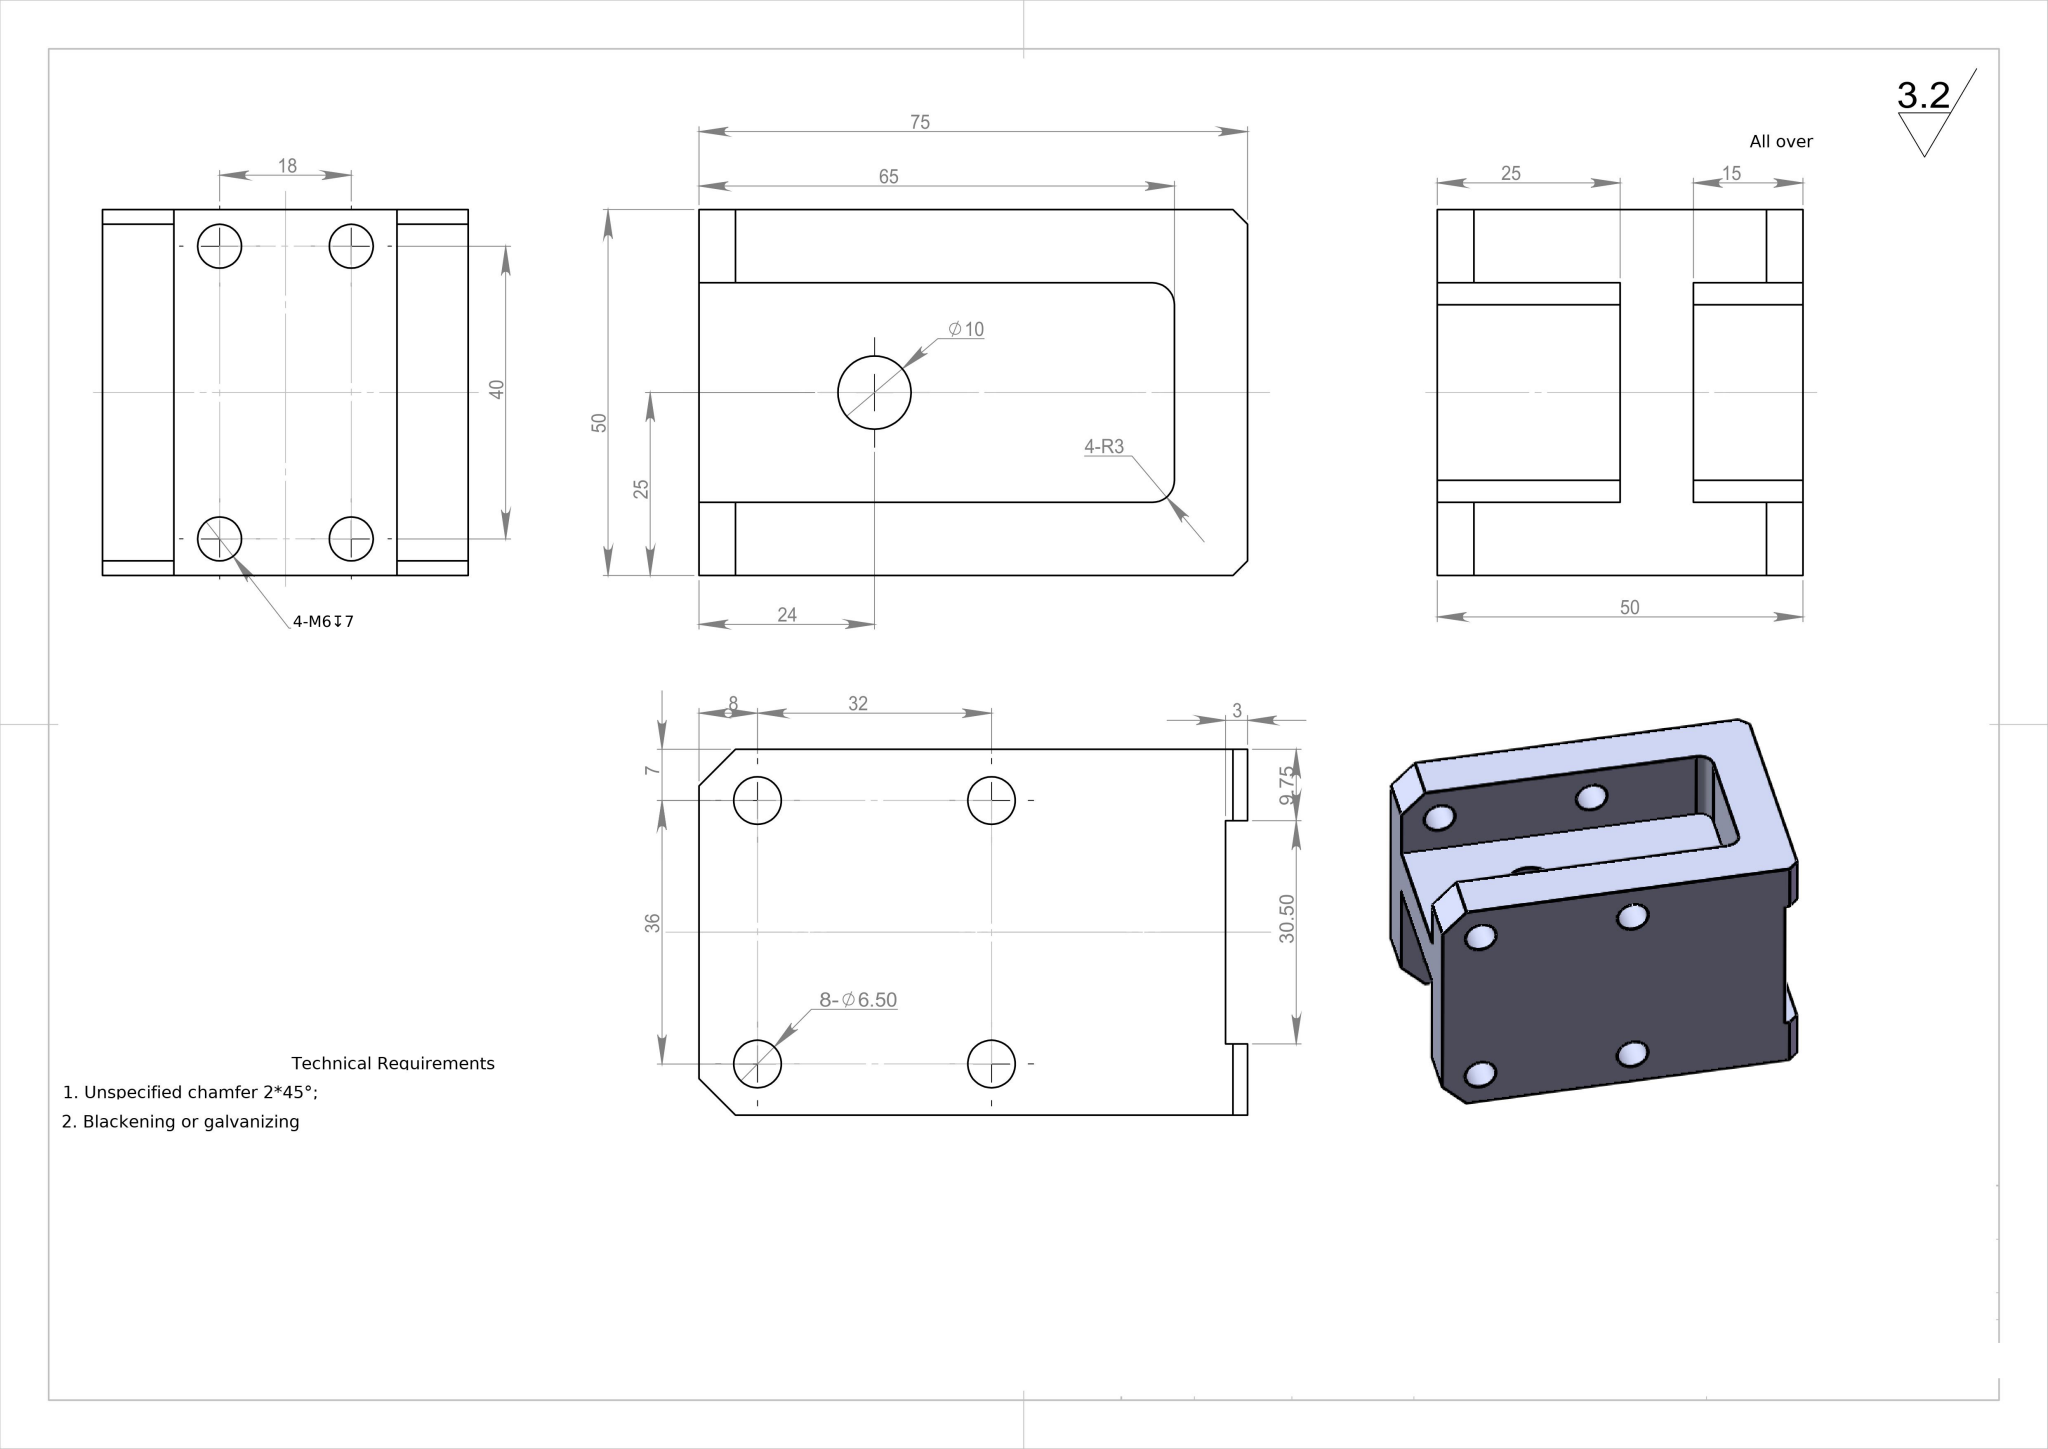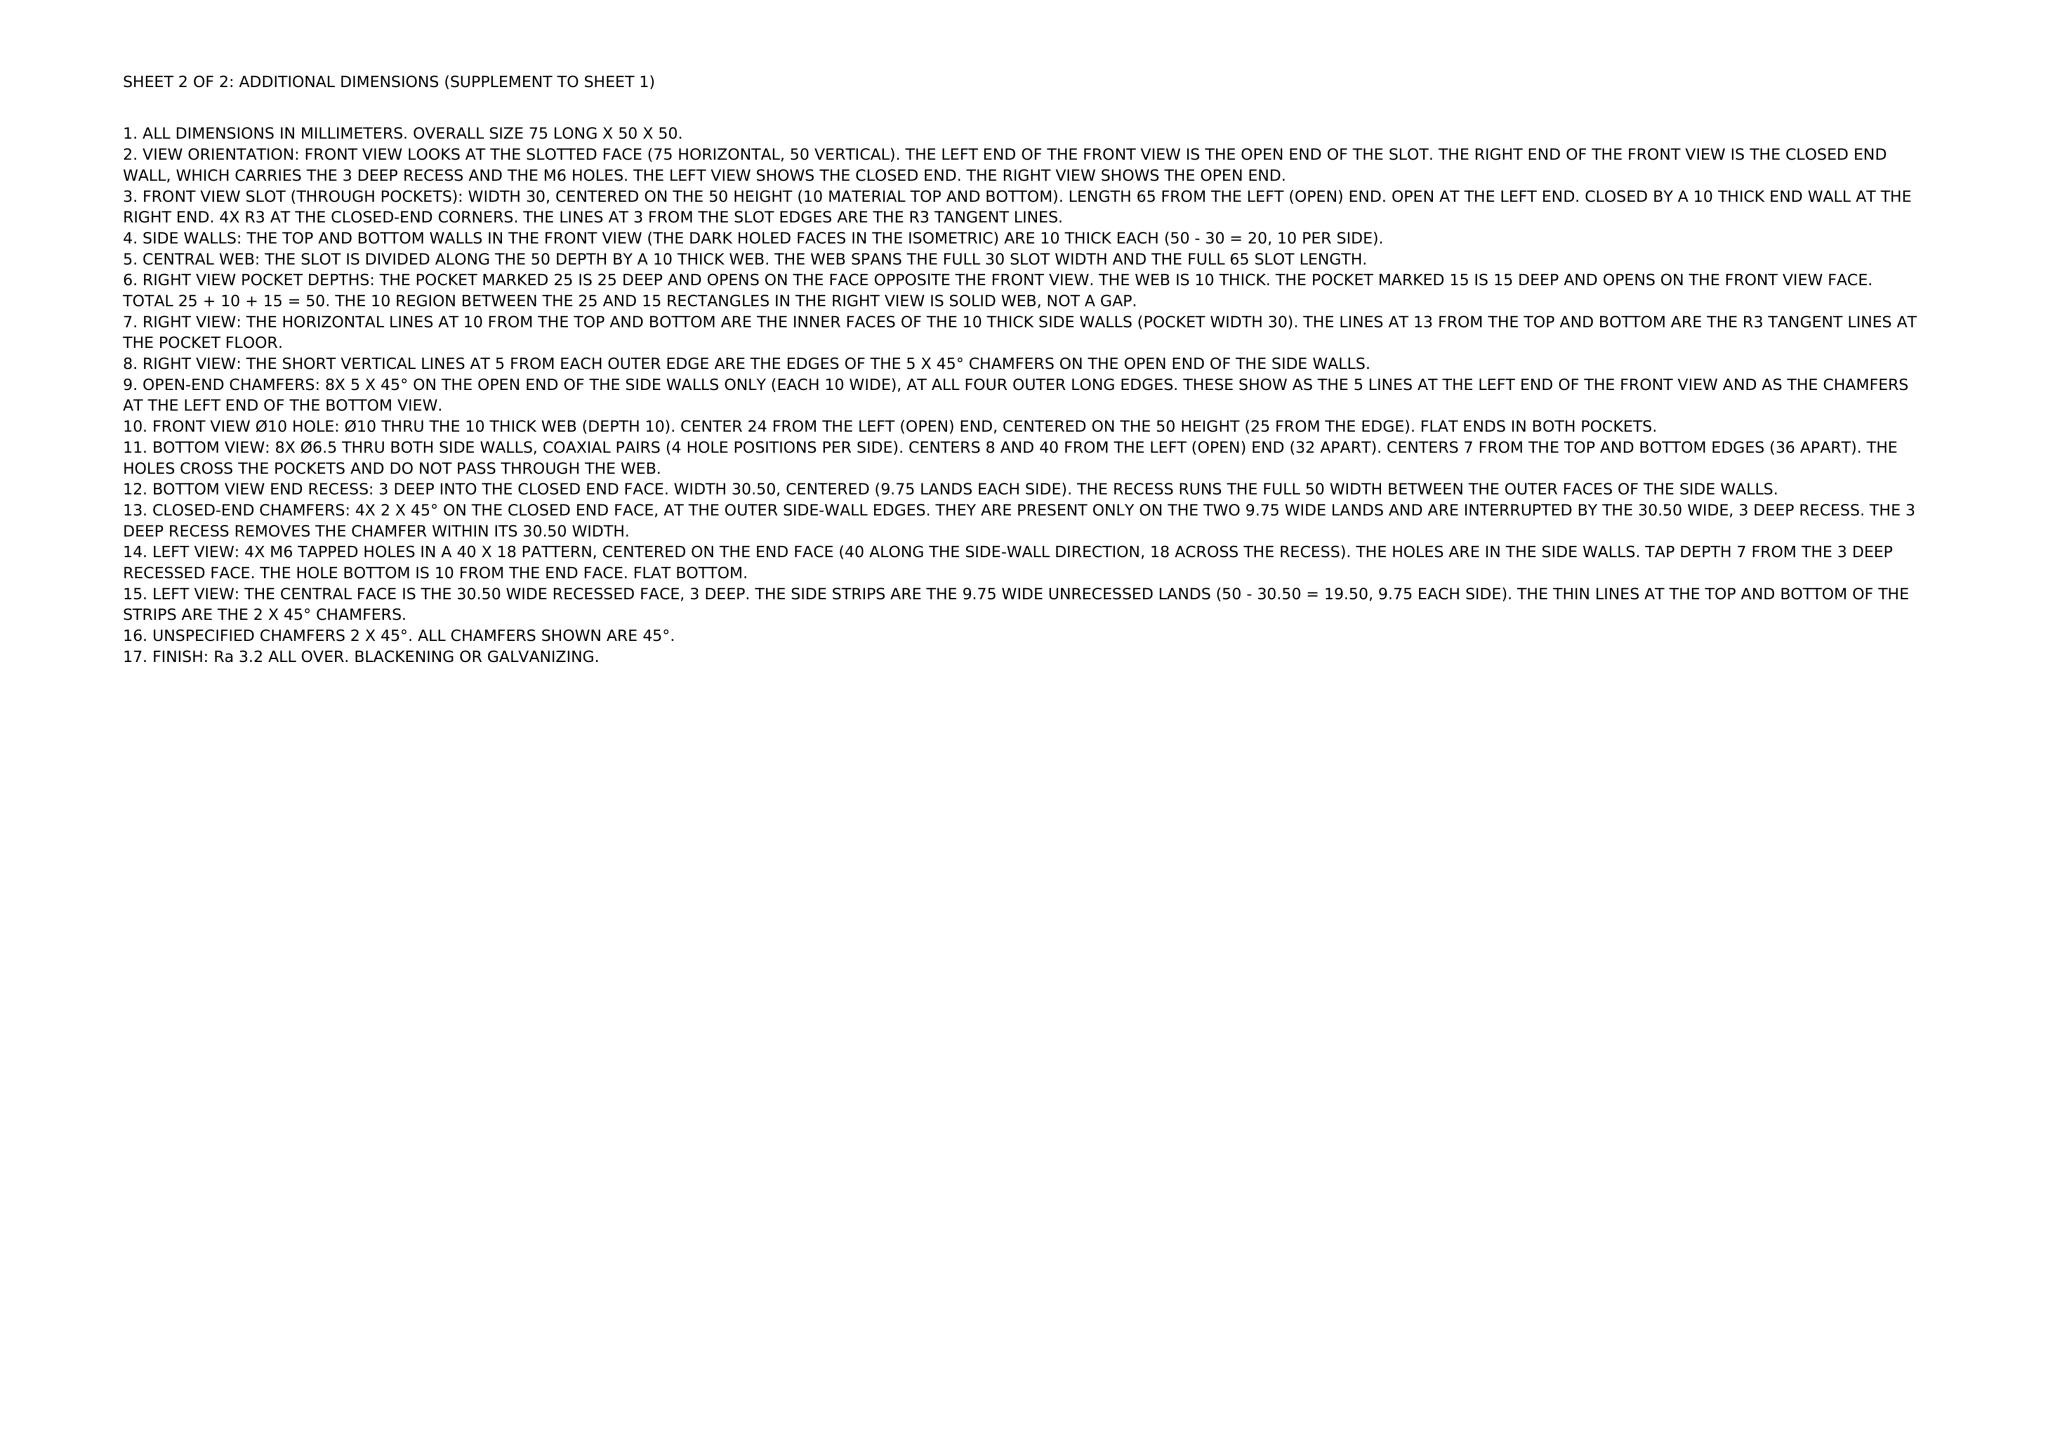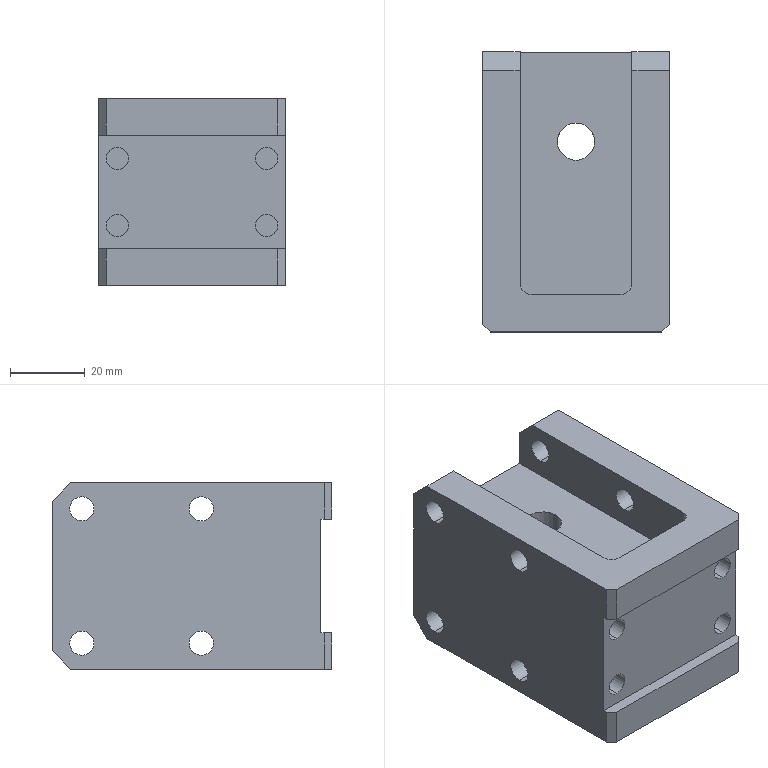Part | NX | mm | 1 solid | 60 faces | box 50 x 75 x 50 mm | volume 100270 mm3 | cylinder 30 | plane 30 | commonest cylinder face diameters 6.5 x16 6 x12 10 x2